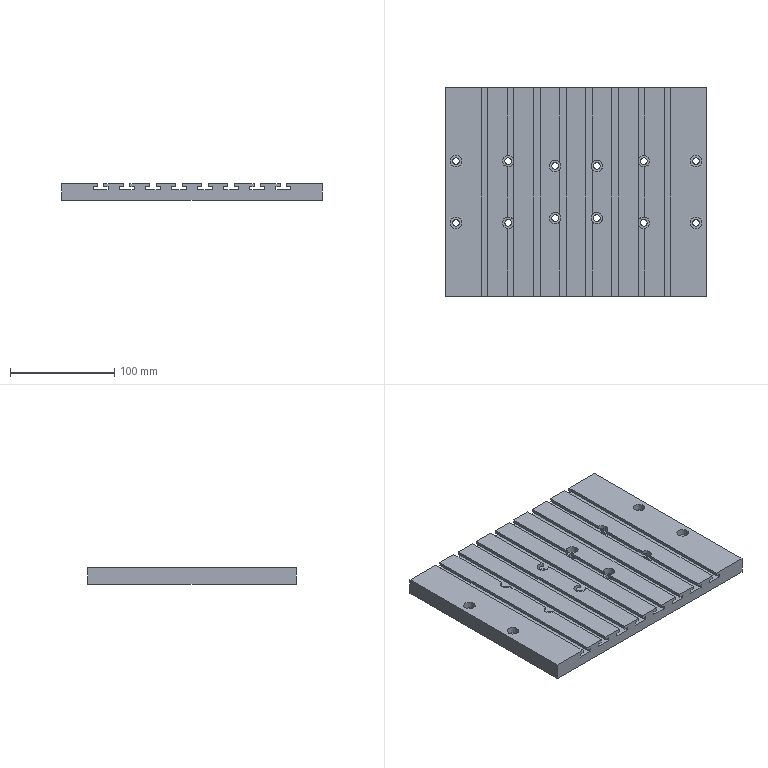Component | NX | WORKBENCH | 1 solid | 134 faces | volume 695276 mm3 | plane 106 | cylinder 28 | commonest cylinder face diameters 11 x16 6.4 x12